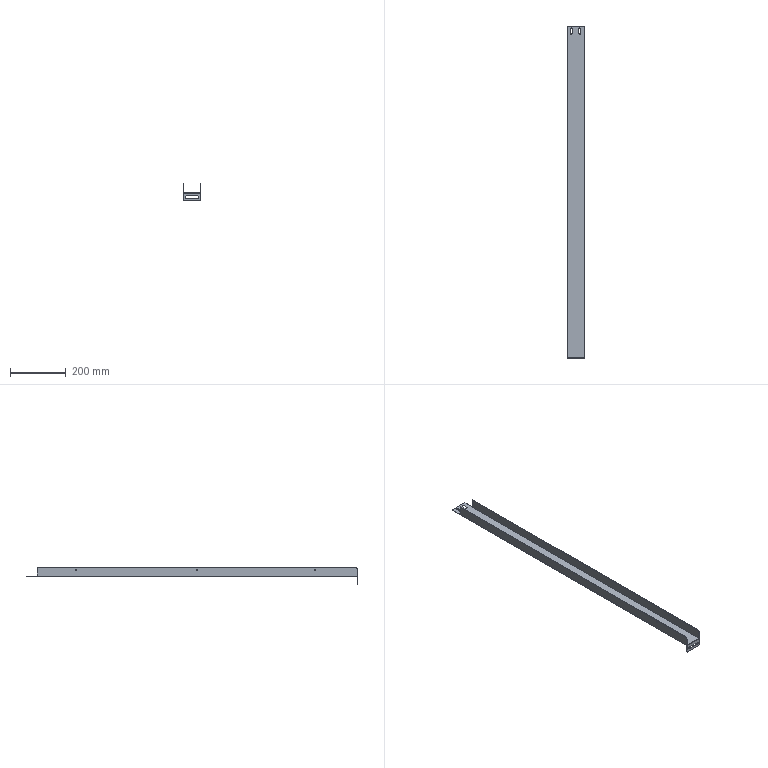Component | SolidWorks | WireDuct1-1 | 1 solid | 45 faces | box 64.11 x 1192 x 62 mm | volume 301711 mm3 | plane 23 | cylinder 22 | commonest cylinder face diameters 4.2 x12 8 x6 20 x2 2 x2
build123d program:
from build123d import *

# Parameters (mm, degrees)
BOSS_EXTRUDE1_DEPTH      = 590
BOSS_EXTRUDE1_DEPTH_BACK = 600
M5_TAPPED_HOLE1_D        = 4.2
FILLET1_R                = 10
SKETCH4_W                = 40
SKETCH4_H                = 40
CUT_EXTRUDE1_DEPTH       = 84
CUT_EXTRUDE2_DEPTH       = 602.814
SKETCH8_W                = 64.112
SKETCH8_H                = 2
BOSS_EXTRUDE3_DEPTH      = 30
FILLET2_R                = 1
CUT_EXTRUDE3_DEPTH       = 30


with BuildPart() as part:
    # Sketch1 → Boss-Extrude1 (new, two sides: drawn at the far end of the back side and taken through both)
    with BuildSketch(Plane(origin=(0, 0, 0), x_dir=(1, 0, 0), z_dir=(0, 1, 0)).offset(-BOSS_EXTRUDE1_DEPTH_BACK)):
        Polygon((32, 17), (32, -17), (-32, -17), (-32, 17), (-30, 17), (-30, 15), (-30, -15), (30, -15), (30, 15), (30, 17), align=None)
    extrude(amount=BOSS_EXTRUDE1_DEPTH + BOSS_EXTRUDE1_DEPTH_BACK)

    # M5 Tapped Hole1 (through all)
    with Locations(Plane.ZY.offset(32)):
        with Locations((-9, -448.324), (-9, -25), (-9, 410.363)):
            Hole(M5_TAPPED_HOLE1_D / 2)

    # Fillet1
    fillet1_edges = [part.edges().sort_by_distance(p)[0] for p in [
        (-31, -600, -17),
        (31, -600, -17),
        (-31, 590, -17),
        (31, 590, -17),
    ]]
    fillet(fillet1_edges, radius=FILLET1_R)

    # Sketch4 → Cut-Extrude1 (cut)
    with BuildSketch(Plane.ZY.offset(32)):
        with Locations((-5, 570)):
            Rectangle(SKETCH4_W, SKETCH4_H)
    extrude(amount=-CUT_EXTRUDE1_DEPTH, mode=Mode.SUBTRACT)

    # Sketch5 → Cut-Extrude2 (cut, through all)
    with BuildSketch(Plane.XY.offset(17)):
        with BuildLine():
            Line((-9, 579.02), (-9, 564.57))
            ThreePointArc((-9, 564.57), (-13, 560.57), (-17, 564.57))
            Line((-17, 564.57), (-17, 579.02))
            ThreePointArc((-17, 579.02), (-13, 583.02), (-9, 579.02))
        make_face()
        with BuildLine():
            Line((21, 579.02), (21, 564.57))
            ThreePointArc((21, 564.57), (17, 560.57), (13, 564.57))
            Line((13, 564.57), (13, 579.02))
            ThreePointArc((13, 579.02), (17, 583.02), (21, 579.02))
        make_face()
    extrude(amount=-CUT_EXTRUDE2_DEPTH, mode=Mode.SUBTRACT)

    # Sketch8 → Boss-Extrude3 (add)
    with BuildSketch(Plane(origin=(0, 0, 15), x_dir=(-1, 0, 0), z_dir=(0, 0, -1))):
        with Locations((-0.05612, -601)):
            Rectangle(SKETCH8_W, SKETCH8_H)
    extrude(amount=-BOSS_EXTRUDE3_DEPTH)

    # Fillet2
    fillet2_edges = [part.edges().sort_by_distance(p)[0] for p in [
        (0.05612, -602, 15),
        (0, -600, 17),
    ]]
    fillet(fillet2_edges, radius=FILLET2_R)

    # Sketch9 → Cut-Extrude3 (cut)
    with BuildSketch(Plane(origin=(0, -600, 0), x_dir=(1, 0, 0), z_dir=(0, 1, 0))):
        with BuildLine():
            Line((-19.944, -28.132), (20.056, -28.132))
            ThreePointArc((20.056, -28.132), (24.056, -32.132), (20.056, -36.132))
            Line((20.056, -36.132), (-19.944, -36.132))
            ThreePointArc((-19.944, -36.132), (-23.944, -32.132), (-19.944, -28.132))
        make_face()
    extrude(amount=-CUT_EXTRUDE3_DEPTH, mode=Mode.SUBTRACT)


solid = part.part

# Placed as in the assembly
solid = solid.moved(Location((613, 1520, -2120), (-180, 0, 180)))